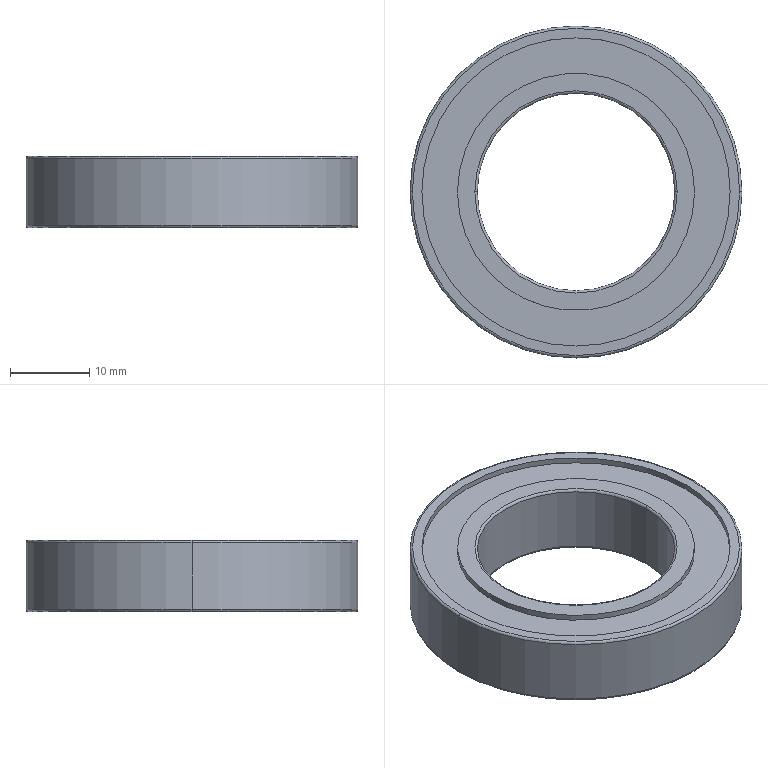Component | SolidWorks | BGRRB6905ZZ-1_bearingB6905ZZ-1 | 1 solid | 26 faces | box 42 x 42 x 9 mm | volume 7311 mm3 | cylinder 12 | torus 8 | plane 6 | commonest cylinder face diameters 39 x4 30 x4 42 x2 25 x2 | material AISI 1045 Steel, cold drawn
build123d program:
from build123d import *


with BuildPart() as part:
    # Sketch1 → Revolve1 (revolve)
    with BuildSketch(Plane.XY, mode=Mode.PRIVATE) as revolve1_sk:
        with BuildLine():
            Line((0, 20.7), (0, 19.5))
            Line((0, 19.5), (0.75, 19.5))
            Line((0.75, 19.5), (0.75, 15))
            Line((0.75, 15), (0, 15))
            Line((0, 15), (0, 12.8))
            ThreePointArc((0, 12.8), (0.08787, 12.588), (0.3, 12.5))
            Line((0.3, 12.5), (8.7, 12.5))
            ThreePointArc((8.7, 12.5), (8.912, 12.588), (9, 12.8))
            Line((9, 12.8), (9, 15))
            Line((9, 15), (8.25, 15))
            Line((8.25, 15), (8.25, 19.5))
            Line((8.25, 19.5), (9, 19.5))
            Line((9, 19.5), (9, 20.7))
            ThreePointArc((9, 20.7), (8.912, 20.912), (8.7, 21))
            Line((8.7, 21), (0.3, 21))
            ThreePointArc((0.3, 21), (0.08787, 20.912), (0, 20.7))
        make_face()
    revolve(revolve1_sk.sketch.rotate(Axis((9, 0, 0), (-1, 0, 0)), 270), axis=Axis((9, 0, 0), (-1, 0, 0)))


solid = part.part

# Placed as in the assembly
solid = solid.moved(Location((0, 0, 69), (0, 90, 0)))
STEP:
#1=COLOUR_RGB('',0.7922,0.8196,0.9333);
#2=FILL_AREA_STYLE_COLOUR('',#1);
#3=FILL_AREA_STYLE('',(#2));
#4=SURFACE_STYLE_FILL_AREA(#3);
#5=SURFACE_SIDE_STYLE('',(#4));
#6=SURFACE_STYLE_USAGE(.BOTH.,#5);
#7=PRESENTATION_STYLE_ASSIGNMENT((#6));
#8=CARTESIAN_POINT('',(-0.8268,0.,2.705));
#9=VERTEX_POINT('',#8);
#10=CARTESIAN_POINT('',(0.8268,0.,2.705));
#11=VERTEX_POINT('',#10);
#12=CARTESIAN_POINT('',(0.,0.,2.705));
#13=DIRECTION('',(0.,0.,-1.));
#14=DIRECTION('',(-1.,-0.,-0.));
#15=AXIS2_PLACEMENT_3D('',#12,#13,#14);
#16=CIRCLE('',#15,0.8268);
#17=EDGE_CURVE('',#9,#11,#16,.T.);
#18=ORIENTED_EDGE('',*,*,#17,.T.);
#19=CARTESIAN_POINT('',(0.8268,0.,2.374));
#20=VERTEX_POINT('',#19);
#21=CARTESIAN_POINT('',(0.8268,0.,2.717));
#22=DIRECTION('',(0.,0.,-1.));
#23=VECTOR('',#22,39.37);
#24=LINE('',#21,#23);
#25=EDGE_CURVE('',#11,#20,#24,.T.);
#26=ORIENTED_EDGE('',*,*,#25,.T.);
#27=CARTESIAN_POINT('',(-0.8268,0.,2.374));
#28=VERTEX_POINT('',#27);
#29=CARTESIAN_POINT('',(0.,0.,2.374));
#30=DIRECTION('',(0.,0.,-1.));
#31=DIRECTION('',(-1.,-0.,-0.));
#32=AXIS2_PLACEMENT_3D('',#29,#30,#31);
#33=CIRCLE('',#32,0.8268);
#34=EDGE_CURVE('',#28,#20,#33,.T.);
#35=ORIENTED_EDGE('',*,*,#34,.F.);
#36=CARTESIAN_POINT('',(-0.8268,0.,2.717));
#37=DIRECTION('',(0.,0.,-1.));
#38=VECTOR('',#37,39.37);
#39=LINE('',#36,#38);
#40=EDGE_CURVE('',#9,#28,#39,.T.);
#41=ORIENTED_EDGE('',*,*,#40,.F.);
#42=EDGE_LOOP('',(#18,#26,#35,#41));
#43=FACE_OUTER_BOUND('',#42,.T.);
#44=CARTESIAN_POINT('',(0.,0.,2.717));
#45=DIRECTION('',(0.,0.,-1.));
#46=DIRECTION('',(-1.,-0.,-0.));
#47=AXIS2_PLACEMENT_3D('',#44,#45,#46);
#48=CYLINDRICAL_SURFACE('',#47,0.8268);
#49=ADVANCED_FACE('',(#43),#48,.T.);
#50=CARTESIAN_POINT('',(-0.815,0.,2.717));
#51=VERTEX_POINT('',#50);
#52=CARTESIAN_POINT('',(0.815,0.,2.717));
#53=VERTEX_POINT('',#52);
#54=CARTESIAN_POINT('',(0.,0.,2.717));
#55=DIRECTION('',(0.,0.,-1.));
#56=DIRECTION('',(-1.,-0.,-0.));
#57=AXIS2_PLACEMENT_3D('',#54,#55,#56);
#58=CIRCLE('',#57,0.815);
#59=EDGE_CURVE('',#51,#53,#58,.T.);
#60=ORIENTED_EDGE('',*,*,#59,.T.);
#61=CARTESIAN_POINT('',(0.815,0.,2.705));
#62=DIRECTION('',(-0.,1.,0.));
#63=DIRECTION('',(-1.,-0.,0.));
#64=AXIS2_PLACEMENT_3D('',#61,#62,#63);
#65=CIRCLE('',#64,0.01181);
#66=EDGE_CURVE('',#53,#11,#65,.T.);
#67=ORIENTED_EDGE('',*,*,#66,.T.);
#68=ORIENTED_EDGE('',*,*,#17,.F.);
#69=CARTESIAN_POINT('',(-0.815,0.,2.705));
#70=DIRECTION('',(0.,-1.,-0.));
#71=DIRECTION('',(1.,0.,0.));
#72=AXIS2_PLACEMENT_3D('',#69,#70,#71);
#73=CIRCLE('',#72,0.01181);
#74=EDGE_CURVE('',#51,#9,#73,.T.);
#75=ORIENTED_EDGE('',*,*,#74,.F.);
#76=EDGE_LOOP('',(#60,#67,#68,#75));
#77=FACE_OUTER_BOUND('',#76,.T.);
#78=CARTESIAN_POINT('',(0.,0.,2.705));
#79=DIRECTION('',(0.,0.,-1.));
#80=DIRECTION('',(-1.,-0.,-0.));
#81=AXIS2_PLACEMENT_3D('',#78,#79,#80);
#82=TOROIDAL_SURFACE('',#81,0.815,0.01181);
#83=ADVANCED_FACE('',(#77),#82,.T.);
#84=CARTESIAN_POINT('',(0.7677,0.,2.717));
#85=VERTEX_POINT('',#84);
#86=CARTESIAN_POINT('',(-0.7677,0.,2.717));
#87=VERTEX_POINT('',#86);
#88=CARTESIAN_POINT('',(0.,0.,2.717));
#89=DIRECTION('',(0.,0.,-1.));
#90=DIRECTION('',(-1.,-0.,-0.));
#91=AXIS2_PLACEMENT_3D('',#88,#89,#90);
#92=CIRCLE('',#91,0.7677);
#93=EDGE_CURVE('',#85,#87,#92,.T.);
#94=ORIENTED_EDGE('',*,*,#93,.F.);
#95=CARTESIAN_POINT('',(0.7677,0.,2.687));
#96=VERTEX_POINT('',#95);
#97=CARTESIAN_POINT('',(0.7677,0.,2.717));
#98=DIRECTION('',(0.,0.,-1.));
#99=VECTOR('',#98,39.37);
#100=LINE('',#97,#99);
#101=EDGE_CURVE('',#85,#96,#100,.T.);
#102=ORIENTED_EDGE('',*,*,#101,.T.);
#103=CARTESIAN_POINT('',(-0.7677,0.,2.687));
#104=VERTEX_POINT('',#103);
#105=CARTESIAN_POINT('',(0.,0.,2.687));
#106=DIRECTION('',(0.,0.,-1.));
#107=DIRECTION('',(-1.,-0.,-0.));
#108=AXIS2_PLACEMENT_3D('',#105,#106,#107);
#109=CIRCLE('',#108,0.7677);
#110=EDGE_CURVE('',#96,#104,#109,.T.);
#111=ORIENTED_EDGE('',*,*,#110,.T.);
#112=CARTESIAN_POINT('',(-0.7677,0.,2.717));
#113=DIRECTION('',(0.,0.,-1.));
#114=VECTOR('',#113,39.37);
#115=LINE('',#112,#114);
#116=EDGE_CURVE('',#87,#104,#115,.T.);
#117=ORIENTED_EDGE('',*,*,#116,.F.);
#118=EDGE_LOOP('',(#94,#102,#111,#117));
#119=FACE_OUTER_BOUND('',#118,.T.);
#120=CARTESIAN_POINT('',(0.,0.,2.717));
#121=DIRECTION('',(0.,0.,-1.));
#122=DIRECTION('',(-1.,-0.,-0.));
#123=AXIS2_PLACEMENT_3D('',#120,#121,#122);
#124=CYLINDRICAL_SURFACE('',#123,0.7677);
#125=ADVANCED_FACE('',(#119),#124,.F.);
#126=CARTESIAN_POINT('',(-0.5906,0.,2.717));
#127=VERTEX_POINT('',#126);
#128=CARTESIAN_POINT('',(0.5906,0.,2.717));
#129=VERTEX_POINT('',#128);
#130=CARTESIAN_POINT('',(0.,0.,2.717));
#131=DIRECTION('',(0.,0.,-1.));
#132=DIRECTION('',(-1.,-0.,0.));
#133=AXIS2_PLACEMENT_3D('',#130,#131,#132);
#134=CIRCLE('',#133,0.5906);
#135=EDGE_CURVE('',#127,#129,#134,.T.);
#136=ORIENTED_EDGE('',*,*,#135,.T.);
#137=CARTESIAN_POINT('',(0.5906,0.,2.687));
#138=VERTEX_POINT('',#137);
#139=CARTESIAN_POINT('',(0.5906,0.,2.717));
#140=DIRECTION('',(0.,0.,-1.));
#141=VECTOR('',#140,39.37);
#142=LINE('',#139,#141);
#143=EDGE_CURVE('',#129,#138,#142,.T.);
#144=ORIENTED_EDGE('',*,*,#143,.T.);
#145=CARTESIAN_POINT('',(-0.5906,0.,2.687));
#146=VERTEX_POINT('',#145);
#147=CARTESIAN_POINT('',(0.,0.,2.687));
#148=DIRECTION('',(0.,0.,-1.));
#149=DIRECTION('',(-1.,-0.,0.));
#150=AXIS2_PLACEMENT_3D('',#147,#148,#149);
#151=CIRCLE('',#150,0.5906);
#152=EDGE_CURVE('',#146,#138,#151,.T.);
#153=ORIENTED_EDGE('',*,*,#152,.F.);
#154=CARTESIAN_POINT('',(-0.5906,0.,2.717));
#155=DIRECTION('',(0.,0.,-1.));
#156=VECTOR('',#155,39.37);
#157=LINE('',#154,#156);
#158=EDGE_CURVE('',#127,#146,#157,.T.);
#159=ORIENTED_EDGE('',*,*,#158,.F.);
#160=EDGE_LOOP('',(#136,#144,#153,#159));
#161=FACE_OUTER_BOUND('',#160,.T.);
#162=CARTESIAN_POINT('',(0.,0.,2.717));
#163=DIRECTION('',(0.,0.,-1.));
#164=DIRECTION('',(-1.,-0.,0.));
#165=AXIS2_PLACEMENT_3D('',#162,#163,#164);
#166=CYLINDRICAL_SURFACE('',#165,0.5906);
#167=ADVANCED_FACE('',(#161),#166,.T.);
#168=CARTESIAN_POINT('',(-0.4921,0.,2.705));
#169=VERTEX_POINT('',#168);
#170=CARTESIAN_POINT('',(0.4921,0.,2.705));
#171=VERTEX_POINT('',#170);
#172=CARTESIAN_POINT('',(0.,0.,2.705));
#173=DIRECTION('',(0.,0.,-1.));
#174=DIRECTION('',(-1.,-0.,0.));
#175=AXIS2_PLACEMENT_3D('',#172,#173,#174);
#176=CIRCLE('',#175,0.4921);
#177=EDGE_CURVE('',#169,#171,#176,.T.);
#178=ORIENTED_EDGE('',*,*,#177,.T.);
#179=CARTESIAN_POINT('',(0.5039,0.,2.717));
#180=VERTEX_POINT('',#179);
#181=CARTESIAN_POINT('',(0.5039,0.,2.705));
#182=DIRECTION('',(-0.,1.,0.));
#183=DIRECTION('',(-1.,-0.,0.));
#184=AXIS2_PLACEMENT_3D('',#181,#182,#183);
#185=CIRCLE('',#184,0.01181);
#186=EDGE_CURVE('',#171,#180,#185,.T.);
#187=ORIENTED_EDGE('',*,*,#186,.T.);
#188=CARTESIAN_POINT('',(-0.5039,0.,2.717));
#189=VERTEX_POINT('',#188);
#190=CARTESIAN_POINT('',(0.,0.,2.717));
#191=DIRECTION('',(0.,0.,-1.));
#192=DIRECTION('',(-1.,-0.,0.));
#193=AXIS2_PLACEMENT_3D('',#190,#191,#192);
#194=CIRCLE('',#193,0.5039);
#195=EDGE_CURVE('',#189,#180,#194,.T.);
#196=ORIENTED_EDGE('',*,*,#195,.F.);
#197=CARTESIAN_POINT('',(-0.5039,0.,2.705));
#198=DIRECTION('',(0.,-1.,-0.));
#199=DIRECTION('',(1.,0.,0.));
#200=AXIS2_PLACEMENT_3D('',#197,#198,#199);
#201=CIRCLE('',#200,0.01181);
#202=EDGE_CURVE('',#169,#189,#201,.T.);
#203=ORIENTED_EDGE('',*,*,#202,.F.);
#204=EDGE_LOOP('',(#178,#187,#196,#203));
#205=FACE_OUTER_BOUND('',#204,.T.);
#206=CARTESIAN_POINT('',(0.,0.,2.705));
#207=DIRECTION('',(0.,0.,-1.));
#208=DIRECTION('',(-1.,-0.,-0.));
#209=AXIS2_PLACEMENT_3D('',#206,#207,#208);
#210=TOROIDAL_SURFACE('',#209,0.5039,0.01181);
#211=ADVANCED_FACE('',(#205),#210,.T.);
#212=CARTESIAN_POINT('',(0.,0.,2.705));
#213=DIRECTION('',(0.,0.,-1.));
#214=DIRECTION('',(-1.,-0.,0.));
#215=AXIS2_PLACEMENT_3D('',#212,#213,#214);
#216=CIRCLE('',#215,0.4921);
#217=EDGE_CURVE('',#171,#169,#216,.T.);
#218=ORIENTED_EDGE('',*,*,#217,.F.);
#219=CARTESIAN_POINT('',(0.4921,0.,2.374));
#220=VERTEX_POINT('',#219);
#221=CARTESIAN_POINT('',(0.4921,0.,2.717));
#222=DIRECTION('',(0.,0.,-1.));
#223=VECTOR('',#222,39.37);
#224=LINE('',#221,#223);
#225=EDGE_CURVE('',#171,#220,#224,.T.);
#226=ORIENTED_EDGE('',*,*,#225,.T.);
#227=CARTESIAN_POINT('',(-0.4921,0.,2.374));
#228=VERTEX_POINT('',#227);
#229=CARTESIAN_POINT('',(0.,0.,2.374));
#230=DIRECTION('',(0.,0.,-1.));
#231=DIRECTION('',(-1.,-0.,-0.));
#232=AXIS2_PLACEMENT_3D('',#229,#230,#231);
#233=CIRCLE('',#232,0.4921);
#234=EDGE_CURVE('',#220,#228,#233,.T.);
#235=ORIENTED_EDGE('',*,*,#234,.T.);
#236=CARTESIAN_POINT('',(-0.4921,0.,2.717));
#237=DIRECTION('',(0.,0.,-1.));
#238=VECTOR('',#237,39.37);
#239=LINE('',#236,#238);
#240=EDGE_CURVE('',#169,#228,#239,.T.);
#241=ORIENTED_EDGE('',*,*,#240,.F.);
#242=EDGE_LOOP('',(#218,#226,#235,#241));
#243=FACE_OUTER_BOUND('',#242,.T.);
#244=CARTESIAN_POINT('',(0.,0.,2.717));
#245=DIRECTION('',(0.,0.,-1.));
#246=DIRECTION('',(-1.,-0.,0.));
#247=AXIS2_PLACEMENT_3D('',#244,#245,#246);
#248=CYLINDRICAL_SURFACE('',#247,0.4921);
#249=ADVANCED_FACE('',(#243),#248,.F.);
#250=CARTESIAN_POINT('',(-0.5039,0.,2.362));
#251=VERTEX_POINT('',#250);
#252=CARTESIAN_POINT('',(0.5039,0.,2.362));
#253=VERTEX_POINT('',#252);
#254=CARTESIAN_POINT('',(0.,0.,2.362));
#255=DIRECTION('',(0.,0.,-1.));
#256=DIRECTION('',(-1.,-0.,-0.));
#257=AXIS2_PLACEMENT_3D('',#254,#255,#256);
#258=CIRCLE('',#257,0.5039);
#259=EDGE_CURVE('',#251,#253,#258,.T.);
#260=ORIENTED_EDGE('',*,*,#259,.T.);
#261=CARTESIAN_POINT('',(0.5039,0.,2.374));
#262=DIRECTION('',(-0.,1.,0.));
#263=DIRECTION('',(-1.,-0.,0.));
#264=AXIS2_PLACEMENT_3D('',#261,#262,#263);
#265=CIRCLE('',#264,0.01181);
#266=EDGE_CURVE('',#253,#220,#265,.T.);
#267=ORIENTED_EDGE('',*,*,#266,.T.);
#268=CARTESIAN_POINT('',(0.,0.,2.374));
#269=DIRECTION('',(0.,0.,-1.));
#270=DIRECTION('',(-1.,-0.,-0.));
#271=AXIS2_PLACEMENT_3D('',#268,#269,#270);
#272=CIRCLE('',#271,0.4921);
#273=EDGE_CURVE('',#228,#220,#272,.T.);
#274=ORIENTED_EDGE('',*,*,#273,.F.);
#275=CARTESIAN_POINT('',(-0.5039,0.,2.374));
#276=DIRECTION('',(0.,-1.,-0.));
#277=DIRECTION('',(1.,0.,0.));
#278=AXIS2_PLACEMENT_3D('',#275,#276,#277);
#279=CIRCLE('',#278,0.01181);
#280=EDGE_CURVE('',#251,#228,#279,.T.);
#281=ORIENTED_EDGE('',*,*,#280,.F.);
#282=EDGE_LOOP('',(#260,#267,#274,#281));
#283=FACE_OUTER_BOUND('',#282,.T.);
#284=CARTESIAN_POINT('',(0.,0.,2.374));
#285=DIRECTION('',(0.,0.,-1.));
#286=DIRECTION('',(-1.,-0.,-0.));
#287=AXIS2_PLACEMENT_3D('',#284,#285,#286);
#288=TOROIDAL_SURFACE('',#287,0.5039,0.01181);
#289=ADVANCED_FACE('',(#283),#288,.T.);
#290=CARTESIAN_POINT('',(-0.5906,0.,2.392));
#291=VERTEX_POINT('',#290);
#292=CARTESIAN_POINT('',(0.5906,0.,2.392));
#293=VERTEX_POINT('',#292);
#294=CARTESIAN_POINT('',(0.,0.,2.392));
#295=DIRECTION('',(0.,0.,-1.));
#296=DIRECTION('',(-1.,-0.,-0.));
#297=AXIS2_PLACEMENT_3D('',#294,#295,#296);
#298=CIRCLE('',#297,0.5906);
#299=EDGE_CURVE('',#291,#293,#298,.T.);
#300=ORIENTED_EDGE('',*,*,#299,.T.);
#301=CARTESIAN_POINT('',(0.5906,0.,2.362));
#302=VERTEX_POINT('',#301);
#303=CARTESIAN_POINT('',(0.5906,0.,2.717));
#304=DIRECTION('',(0.,0.,-1.));
#305=VECTOR('',#304,39.37);
#306=LINE('',#303,#305);
#307=EDGE_CURVE('',#293,#302,#306,.T.);
#308=ORIENTED_EDGE('',*,*,#307,.T.);
#309=CARTESIAN_POINT('',(-0.5906,0.,2.362));
#310=VERTEX_POINT('',#309);
#311=CARTESIAN_POINT('',(0.,0.,2.362));
#312=DIRECTION('',(0.,0.,-1.));
#313=DIRECTION('',(-1.,-0.,-0.));
#314=AXIS2_PLACEMENT_3D('',#311,#312,#313);
#315=CIRCLE('',#314,0.5906);
#316=EDGE_CURVE('',#310,#302,#315,.T.);
#317=ORIENTED_EDGE('',*,*,#316,.F.);
#318=CARTESIAN_POINT('',(-0.5906,0.,2.717));
#319=DIRECTION('',(0.,0.,-1.));
#320=VECTOR('',#319,39.37);
#321=LINE('',#318,#320);
#322=EDGE_CURVE('',#291,#310,#321,.T.);
#323=ORIENTED_EDGE('',*,*,#322,.F.);
#324=EDGE_LOOP('',(#300,#308,#317,#323));
#325=FACE_OUTER_BOUND('',#324,.T.);
#326=CARTESIAN_POINT('',(0.,0.,2.717));
#327=DIRECTION('',(0.,0.,-1.));
#328=DIRECTION('',(-1.,-0.,0.));
#329=AXIS2_PLACEMENT_3D('',#326,#327,#328);
#330=CYLINDRICAL_SURFACE('',#329,0.5906);
#331=ADVANCED_FACE('',(#325),#330,.T.);
#332=CARTESIAN_POINT('',(0.7677,0.,2.392));
#333=VERTEX_POINT('',#332);
#334=CARTESIAN_POINT('',(-0.7677,0.,2.392));
#335=VERTEX_POINT('',#334);
#336=CARTESIAN_POINT('',(0.,0.,2.392));
#337=DIRECTION('',(0.,0.,-1.));
#338=DIRECTION('',(-1.,-0.,-0.));
#339=AXIS2_PLACEMENT_3D('',#336,#337,#338);
#340=CIRCLE('',#339,0.7677);
#341=EDGE_CURVE('',#333,#335,#340,.T.);
#342=ORIENTED_EDGE('',*,*,#341,.F.);
#343=CARTESIAN_POINT('',(0.7677,0.,2.362));
#344=VERTEX_POINT('',#343);
#345=CARTESIAN_POINT('',(0.7677,0.,2.717));
#346=DIRECTION('',(0.,0.,-1.));
#347=VECTOR('',#346,39.37);
#348=LINE('',#345,#347);
#349=EDGE_CURVE('',#333,#344,#348,.T.);
#350=ORIENTED_EDGE('',*,*,#349,.T.);
#351=CARTESIAN_POINT('',(-0.7677,0.,2.362));
#352=VERTEX_POINT('',#351);
#353=CARTESIAN_POINT('',(0.,0.,2.362));
#354=DIRECTION('',(0.,0.,-1.));
#355=DIRECTION('',(-1.,-0.,-0.));
#356=AXIS2_PLACEMENT_3D('',#353,#354,#355);
#357=CIRCLE('',#356,0.7677);
#358=EDGE_CURVE('',#344,#352,#357,.T.);
#359=ORIENTED_EDGE('',*,*,#358,.T.);
#360=CARTESIAN_POINT('',(-0.7677,0.,2.717));
#361=DIRECTION('',(0.,0.,-1.));
#362=VECTOR('',#361,39.37);
#363=LINE('',#360,#362);
#364=EDGE_CURVE('',#335,#352,#363,.T.);
#365=ORIENTED_EDGE('',*,*,#364,.F.);
#366=EDGE_LOOP('',(#342,#350,#359,#365));
#367=FACE_OUTER_BOUND('',#366,.T.);
#368=CARTESIAN_POINT('',(0.,0.,2.717));
#369=DIRECTION('',(0.,0.,-1.));
#370=DIRECTION('',(-1.,-0.,-0.));
#371=AXIS2_PLACEMENT_3D('',#368,#369,#370);
#372=CYLINDRICAL_SURFACE('',#371,0.7677);
#373=ADVANCED_FACE('',(#367),#372,.F.);
#374=ORIENTED_EDGE('',*,*,#34,.T.);
#375=CARTESIAN_POINT('',(0.815,0.,2.362));
#376=VERTEX_POINT('',#375);
#377=CARTESIAN_POINT('',(0.815,0.,2.374));
#378=DIRECTION('',(-0.,1.,0.));
#379=DIRECTION('',(-1.,-0.,0.));
#380=AXIS2_PLACEMENT_3D('',#377,#378,#379);
#381=CIRCLE('',#380,0.01181);
#382=EDGE_CURVE('',#20,#376,#381,.T.);
#383=ORIENTED_EDGE('',*,*,#382,.T.);
#384=CARTESIAN_POINT('',(-0.815,0.,2.362));
#385=VERTEX_POINT('',#384);
#386=CARTESIAN_POINT('',(0.,0.,2.362));
#387=DIRECTION('',(0.,0.,-1.));
#388=DIRECTION('',(-1.,-0.,-0.));
#389=AXIS2_PLACEMENT_3D('',#386,#387,#388);
#390=CIRCLE('',#389,0.815);
#391=EDGE_CURVE('',#385,#376,#390,.T.);
#392=ORIENTED_EDGE('',*,*,#391,.F.);
#393=CARTESIAN_POINT('',(-0.815,0.,2.374));
#394=DIRECTION('',(0.,-1.,-0.));
#395=DIRECTION('',(1.,0.,0.));
#396=AXIS2_PLACEMENT_3D('',#393,#394,#395);
#397=CIRCLE('',#396,0.01181);
#398=EDGE_CURVE('',#28,#385,#397,.T.);
#399=ORIENTED_EDGE('',*,*,#398,.F.);
#400=EDGE_LOOP('',(#374,#383,#392,#399));
#401=FACE_OUTER_BOUND('',#400,.T.);
#402=CARTESIAN_POINT('',(0.,0.,2.374));
#403=DIRECTION('',(0.,0.,-1.));
#404=DIRECTION('',(-1.,-0.,-0.));
#405=AXIS2_PLACEMENT_3D('',#402,#403,#404);
#406=TOROIDAL_SURFACE('',#405,0.815,0.01181);
#407=ADVANCED_FACE('',(#401),#406,.T.);
#408=ORIENTED_EDGE('',*,*,#382,.F.);
#409=CARTESIAN_POINT('',(0.,0.,2.374));
#410=DIRECTION('',(0.,0.,-1.));
#411=DIRECTION('',(-1.,-0.,-0.));
#412=AXIS2_PLACEMENT_3D('',#409,#410,#411);
#413=CIRCLE('',#412,0.8268);
#414=EDGE_CURVE('',#20,#28,#413,.T.);
#415=ORIENTED_EDGE('',*,*,#414,.T.);
#416=ORIENTED_EDGE('',*,*,#398,.T.);
#417=CARTESIAN_POINT('',(0.,0.,2.362));
#418=DIRECTION('',(0.,0.,-1.));
#419=DIRECTION('',(-1.,-0.,-0.));
#420=AXIS2_PLACEMENT_3D('',#417,#418,#419);
#421=CIRCLE('',#420,0.815);
#422=EDGE_CURVE('',#376,#385,#421,.T.);
#423=ORIENTED_EDGE('',*,*,#422,.F.);
#424=EDGE_LOOP('',(#408,#415,#416,#423));
#425=FACE_OUTER_BOUND('',#424,.T.);
#426=CARTESIAN_POINT('',(0.,0.,2.374));
#427=DIRECTION('',(0.,0.,-1.));
#428=DIRECTION('',(-1.,-0.,-0.));
#429=AXIS2_PLACEMENT_3D('',#426,#427,#428);
#430=TOROIDAL_SURFACE('',#429,0.815,0.01181);
#431=ADVANCED_FACE('',(#425),#430,.T.);
#432=CARTESIAN_POINT('',(0.,0.,2.362));
#433=DIRECTION('',(0.,0.,-1.));
#434=DIRECTION('',(-1.,-0.,-0.));
#435=AXIS2_PLACEMENT_3D('',#432,#433,#434);
#436=CIRCLE('',#435,0.7677);
#437=EDGE_CURVE('',#352,#344,#436,.T.);
#438=ORIENTED_EDGE('',*,*,#437,.F.);
#439=ORIENTED_EDGE('',*,*,#358,.F.);
#440=EDGE_LOOP('',(#438,#439));
#441=FACE_BOUND('',#440,.T.);
#442=ORIENTED_EDGE('',*,*,#391,.T.);
#443=ORIENTED_EDGE('',*,*,#422,.T.);
#444=EDGE_LOOP('',(#442,#443));
#445=FACE_OUTER_BOUND('',#444,.T.);
#446=CARTESIAN_POINT('',(0.,0.815,2.362));
#447=DIRECTION('',(-0.,-0.,1.));
#448=DIRECTION('',(1.,0.,0.));
#449=AXIS2_PLACEMENT_3D('',#446,#447,#448);
#450=PLANE('',#449);
#451=ADVANCED_FACE('',(#441,#445),#450,.F.);
#452=ORIENTED_EDGE('',*,*,#349,.F.);
#453=CARTESIAN_POINT('',(0.,0.,2.392));
#454=DIRECTION('',(0.,0.,-1.));
#455=DIRECTION('',(-1.,-0.,-0.));
#456=AXIS2_PLACEMENT_3D('',#453,#454,#455);
#457=CIRCLE('',#456,0.7677);
#458=EDGE_CURVE('',#335,#333,#457,.T.);
#459=ORIENTED_EDGE('',*,*,#458,.F.);
#460=ORIENTED_EDGE('',*,*,#364,.T.);
#461=ORIENTED_EDGE('',*,*,#437,.T.);
#462=EDGE_LOOP('',(#452,#459,#460,#461));
#463=FACE_OUTER_BOUND('',#462,.T.);
#464=CARTESIAN_POINT('',(0.,0.,2.717));
#465=DIRECTION('',(0.,0.,-1.));
#466=DIRECTION('',(-1.,-0.,-0.));
#467=AXIS2_PLACEMENT_3D('',#464,#465,#466);
#468=CYLINDRICAL_SURFACE('',#467,0.7677);
#469=ADVANCED_FACE('',(#463),#468,.F.);
#470=ORIENTED_EDGE('',*,*,#299,.F.);
#471=CARTESIAN_POINT('',(0.,0.,2.392));
#472=DIRECTION('',(0.,0.,-1.));
#473=DIRECTION('',(-1.,-0.,-0.));
#474=AXIS2_PLACEMENT_3D('',#471,#472,#473);
#475=CIRCLE('',#474,0.5906);
#476=EDGE_CURVE('',#293,#291,#475,.T.);
#477=ORIENTED_EDGE('',*,*,#476,.F.);
#478=EDGE_LOOP('',(#470,#477));
#479=FACE_BOUND('',#478,.T.);
#480=ORIENTED_EDGE('',*,*,#458,.T.);
#481=ORIENTED_EDGE('',*,*,#341,.T.);
#482=EDGE_LOOP('',(#480,#481));
#483=FACE_OUTER_BOUND('',#482,.T.);
#484=CARTESIAN_POINT('',(0.,0.7677,2.392));
#485=DIRECTION('',(-0.,-0.,1.));
#486=DIRECTION('',(1.,0.,0.));
#487=AXIS2_PLACEMENT_3D('',#484,#485,#486);
#488=PLANE('',#487);
#489=ADVANCED_FACE('',(#479,#483),#488,.F.);
#490=ORIENTED_EDGE('',*,*,#307,.F.);
#491=ORIENTED_EDGE('',*,*,#476,.T.);
#492=ORIENTED_EDGE('',*,*,#322,.T.);
#493=CARTESIAN_POINT('',(0.,0.,2.362));
#494=DIRECTION('',(0.,0.,-1.));
#495=DIRECTION('',(-1.,-0.,-0.));
#496=AXIS2_PLACEMENT_3D('',#493,#494,#495);
#497=CIRCLE('',#496,0.5906);
#498=EDGE_CURVE('',#302,#310,#497,.T.);
#499=ORIENTED_EDGE('',*,*,#498,.F.);
#500=EDGE_LOOP('',(#490,#491,#492,#499));
#501=FACE_OUTER_BOUND('',#500,.T.);
#502=CARTESIAN_POINT('',(0.,0.,2.717));
#503=DIRECTION('',(0.,0.,-1.));
#504=DIRECTION('',(-1.,-0.,0.));
#505=AXIS2_PLACEMENT_3D('',#502,#503,#504);
#506=CYLINDRICAL_SURFACE('',#505,0.5906);
#507=ADVANCED_FACE('',(#501),#506,.T.);
#508=ORIENTED_EDGE('',*,*,#259,.F.);
#509=CARTESIAN_POINT('',(0.,0.,2.362));
#510=DIRECTION('',(0.,0.,-1.));
#511=DIRECTION('',(-1.,-0.,-0.));
#512=AXIS2_PLACEMENT_3D('',#509,#510,#511);
#513=CIRCLE('',#512,0.5039);
#514=EDGE_CURVE('',#253,#251,#513,.T.);
#515=ORIENTED_EDGE('',*,*,#514,.F.);
#516=EDGE_LOOP('',(#508,#515));
#517=FACE_BOUND('',#516,.T.);
#518=ORIENTED_EDGE('',*,*,#316,.T.);
#519=ORIENTED_EDGE('',*,*,#498,.T.);
#520=EDGE_LOOP('',(#518,#519));
#521=FACE_OUTER_BOUND('',#520,.T.);
#522=CARTESIAN_POINT('',(0.,0.5906,2.362));
#523=DIRECTION('',(-0.,-0.,1.));
#524=DIRECTION('',(1.,0.,0.));
#525=AXIS2_PLACEMENT_3D('',#522,#523,#524);
#526=PLANE('',#525);
#527=ADVANCED_FACE('',(#517,#521),#526,.F.);
#528=ORIENTED_EDGE('',*,*,#266,.F.);
#529=ORIENTED_EDGE('',*,*,#514,.T.);
#530=ORIENTED_EDGE('',*,*,#280,.T.);
#531=ORIENTED_EDGE('',*,*,#234,.F.);
#532=EDGE_LOOP('',(#528,#529,#530,#531));
#533=FACE_OUTER_BOUND('',#532,.T.);
#534=CARTESIAN_POINT('',(0.,0.,2.374));
#535=DIRECTION('',(0.,0.,-1.));
#536=DIRECTION('',(-1.,-0.,-0.));
#537=AXIS2_PLACEMENT_3D('',#534,#535,#536);
#538=TOROIDAL_SURFACE('',#537,0.5039,0.01181);
#539=ADVANCED_FACE('',(#533),#538,.T.);
#540=ORIENTED_EDGE('',*,*,#225,.F.);
#541=ORIENTED_EDGE('',*,*,#177,.F.);
#542=ORIENTED_EDGE('',*,*,#240,.T.);
#543=ORIENTED_EDGE('',*,*,#273,.T.);
#544=EDGE_LOOP('',(#540,#541,#542,#543));
#545=FACE_OUTER_BOUND('',#544,.T.);
#546=CARTESIAN_POINT('',(0.,0.,2.717));
#547=DIRECTION('',(0.,0.,-1.));
#548=DIRECTION('',(-1.,-0.,0.));
#549=AXIS2_PLACEMENT_3D('',#546,#547,#548);
#550=CYLINDRICAL_SURFACE('',#549,0.4921);
#551=ADVANCED_FACE('',(#545),#550,.F.);
#552=ORIENTED_EDGE('',*,*,#186,.F.);
#553=ORIENTED_EDGE('',*,*,#217,.T.);
#554=ORIENTED_EDGE('',*,*,#202,.T.);
#555=CARTESIAN_POINT('',(0.,0.,2.717));
#556=DIRECTION('',(0.,0.,-1.));
#557=DIRECTION('',(-1.,-0.,0.));
#558=AXIS2_PLACEMENT_3D('',#555,#556,#557);
#559=CIRCLE('',#558,0.5039);
#560=EDGE_CURVE('',#180,#189,#559,.T.);
#561=ORIENTED_EDGE('',*,*,#560,.F.);
#562=EDGE_LOOP('',(#552,#553,#554,#561));
#563=FACE_OUTER_BOUND('',#562,.T.);
#564=CARTESIAN_POINT('',(0.,0.,2.705));
#565=DIRECTION('',(0.,0.,-1.));
#566=DIRECTION('',(-1.,-0.,-0.));
#567=AXIS2_PLACEMENT_3D('',#564,#565,#566);
#568=TOROIDAL_SURFACE('',#567,0.5039,0.01181);
#569=ADVANCED_FACE('',(#563),#568,.T.);
#570=ORIENTED_EDGE('',*,*,#135,.F.);
#571=CARTESIAN_POINT('',(0.,0.,2.717));
#572=DIRECTION('',(0.,0.,-1.));
#573=DIRECTION('',(-1.,-0.,0.));
#574=AXIS2_PLACEMENT_3D('',#571,#572,#573);
#575=CIRCLE('',#574,0.5906);
#576=EDGE_CURVE('',#129,#127,#575,.T.);
#577=ORIENTED_EDGE('',*,*,#576,.F.);
#578=EDGE_LOOP('',(#570,#577));
#579=FACE_OUTER_BOUND('',#578,.T.);
#580=ORIENTED_EDGE('',*,*,#195,.T.);
#581=ORIENTED_EDGE('',*,*,#560,.T.);
#582=EDGE_LOOP('',(#580,#581));
#583=FACE_BOUND('',#582,.T.);
#584=CARTESIAN_POINT('',(0.,0.5039,2.717));
#585=DIRECTION('',(0.,0.,-1.));
#586=DIRECTION('',(-1.,-0.,-0.));
#587=AXIS2_PLACEMENT_3D('',#584,#585,#586);
#588=PLANE('',#587);
#589=ADVANCED_FACE('',(#579,#583),#588,.F.);
#590=ORIENTED_EDGE('',*,*,#143,.F.);
#591=ORIENTED_EDGE('',*,*,#576,.T.);
#592=ORIENTED_EDGE('',*,*,#158,.T.);
#593=CARTESIAN_POINT('',(0.,0.,2.687));
#594=DIRECTION('',(0.,0.,-1.));
#595=DIRECTION('',(-1.,-0.,0.));
#596=AXIS2_PLACEMENT_3D('',#593,#594,#595);
#597=CIRCLE('',#596,0.5906);
#598=EDGE_CURVE('',#138,#146,#597,.T.);
#599=ORIENTED_EDGE('',*,*,#598,.F.);
#600=EDGE_LOOP('',(#590,#591,#592,#599));
#601=FACE_OUTER_BOUND('',#600,.T.);
#602=CARTESIAN_POINT('',(0.,0.,2.717));
#603=DIRECTION('',(0.,0.,-1.));
#604=DIRECTION('',(-1.,-0.,0.));
#605=AXIS2_PLACEMENT_3D('',#602,#603,#604);
#606=CYLINDRICAL_SURFACE('',#605,0.5906);
#607=ADVANCED_FACE('',(#601),#606,.T.);
#608=CARTESIAN_POINT('',(0.,0.,2.687));
#609=DIRECTION('',(0.,0.,-1.));
#610=DIRECTION('',(-1.,-0.,-0.));
#611=AXIS2_PLACEMENT_3D('',#608,#609,#610);
#612=CIRCLE('',#611,0.7677);
#613=EDGE_CURVE('',#104,#96,#612,.T.);
#614=ORIENTED_EDGE('',*,*,#613,.F.);
#615=ORIENTED_EDGE('',*,*,#110,.F.);
#616=EDGE_LOOP('',(#614,#615));
#617=FACE_OUTER_BOUND('',#616,.T.);
#618=ORIENTED_EDGE('',*,*,#152,.T.);
#619=ORIENTED_EDGE('',*,*,#598,.T.);
#620=EDGE_LOOP('',(#618,#619));
#621=FACE_BOUND('',#620,.T.);
#622=CARTESIAN_POINT('',(0.,0.5906,2.687));
#623=DIRECTION('',(0.,0.,-1.));
#624=DIRECTION('',(-1.,-0.,-0.));
#625=AXIS2_PLACEMENT_3D('',#622,#623,#624);
#626=PLANE('',#625);
#627=ADVANCED_FACE('',(#617,#621),#626,.F.);
#628=ORIENTED_EDGE('',*,*,#101,.F.);
#629=CARTESIAN_POINT('',(0.,0.,2.717));
#630=DIRECTION('',(0.,0.,-1.));
#631=DIRECTION('',(-1.,-0.,-0.));
#632=AXIS2_PLACEMENT_3D('',#629,#630,#631);
#633=CIRCLE('',#632,0.7677);
#634=EDGE_CURVE('',#87,#85,#633,.T.);
#635=ORIENTED_EDGE('',*,*,#634,.F.);
#636=ORIENTED_EDGE('',*,*,#116,.T.);
#637=ORIENTED_EDGE('',*,*,#613,.T.);
#638=EDGE_LOOP('',(#628,#635,#636,#637));
#639=FACE_OUTER_BOUND('',#638,.T.);
#640=CARTESIAN_POINT('',(0.,0.,2.717));
#641=DIRECTION('',(0.,0.,-1.));
#642=DIRECTION('',(-1.,-0.,-0.));
#643=AXIS2_PLACEMENT_3D('',#640,#641,#642);
#644=CYLINDRICAL_SURFACE('',#643,0.7677);
#645=ADVANCED_FACE('',(#639),#644,.F.);
#646=ORIENTED_EDGE('',*,*,#59,.F.);
#647=CARTESIAN_POINT('',(0.,0.,2.717));
#648=DIRECTION('',(0.,0.,-1.));
#649=DIRECTION('',(-1.,-0.,-0.));
#650=AXIS2_PLACEMENT_3D('',#647,#648,#649);
#651=CIRCLE('',#650,0.815);
#652=EDGE_CURVE('',#53,#51,#651,.T.);
#653=ORIENTED_EDGE('',*,*,#652,.F.);
#654=EDGE_LOOP('',(#646,#653));
#655=FACE_OUTER_BOUND('',#654,.T.);
#656=ORIENTED_EDGE('',*,*,#634,.T.);
#657=ORIENTED_EDGE('',*,*,#93,.T.);
#658=EDGE_LOOP('',(#656,#657));
#659=FACE_BOUND('',#658,.T.);
#660=CARTESIAN_POINT('',(0.,0.7677,2.717));
#661=DIRECTION('',(0.,0.,-1.));
#662=DIRECTION('',(-1.,-0.,-0.));
#663=AXIS2_PLACEMENT_3D('',#660,#661,#662);
#664=PLANE('',#663);
#665=ADVANCED_FACE('',(#655,#659),#664,.F.);
#666=ORIENTED_EDGE('',*,*,#66,.F.);
#667=ORIENTED_EDGE('',*,*,#652,.T.);
#668=ORIENTED_EDGE('',*,*,#74,.T.);
#669=CARTESIAN_POINT('',(0.,0.,2.705));
#670=DIRECTION('',(0.,0.,-1.));
#671=DIRECTION('',(-1.,-0.,-0.));
#672=AXIS2_PLACEMENT_3D('',#669,#670,#671);
#673=CIRCLE('',#672,0.8268);
#674=EDGE_CURVE('',#11,#9,#673,.T.);
#675=ORIENTED_EDGE('',*,*,#674,.F.);
#676=EDGE_LOOP('',(#666,#667,#668,#675));
#677=FACE_OUTER_BOUND('',#676,.T.);
#678=CARTESIAN_POINT('',(0.,0.,2.705));
#679=DIRECTION('',(0.,0.,-1.));
#680=DIRECTION('',(-1.,-0.,-0.));
#681=AXIS2_PLACEMENT_3D('',#678,#679,#680);
#682=TOROIDAL_SURFACE('',#681,0.815,0.01181);
#683=ADVANCED_FACE('',(#677),#682,.T.);
#684=ORIENTED_EDGE('',*,*,#25,.F.);
#685=ORIENTED_EDGE('',*,*,#674,.T.);
#686=ORIENTED_EDGE('',*,*,#40,.T.);
#687=ORIENTED_EDGE('',*,*,#414,.F.);
#688=EDGE_LOOP('',(#684,#685,#686,#687));
#689=FACE_OUTER_BOUND('',#688,.T.);
#690=CARTESIAN_POINT('',(0.,0.,2.717));
#691=DIRECTION('',(0.,0.,-1.));
#692=DIRECTION('',(-1.,-0.,-0.));
#693=AXIS2_PLACEMENT_3D('',#690,#691,#692);
#694=CYLINDRICAL_SURFACE('',#693,0.8268);
#695=ADVANCED_FACE('',(#689),#694,.T.);
#696=CLOSED_SHELL('',(#49,#83,#125,#167,#211,#249,#289,#331,#373,#407,#431,#451,#469,#489,#507,#527,#539,#551,#569,#589,#607,#627,#645,#665,#683,#695));
#697=MANIFOLD_SOLID_BREP('',#696);
#698=STYLED_ITEM('',(#7),#697);
#699=PRESENTATION_LAYER_ASSIGNMENT('','',(#698));
#700=(LENGTH_UNIT()NAMED_UNIT(*)SI_UNIT($,.METRE.));
#701=LENGTH_MEASURE_WITH_UNIT(LENGTH_MEASURE(0.0254),#700);
#702=DIMENSIONAL_EXPONENTS(1.,0.,0.,0.,0.,0.,0.);
#703=(CONVERSION_BASED_UNIT('',#701)LENGTH_UNIT()NAMED_UNIT(#702));
#704=UNCERTAINTY_MEASURE_WITH_UNIT(LENGTH_MEASURE(0.00001),#703,'','');
#705=(NAMED_UNIT(*)PLANE_ANGLE_UNIT()SI_UNIT($,.RADIAN.));
#706=(NAMED_UNIT(*)SI_UNIT($,.STERADIAN.)SOLID_ANGLE_UNIT());
#707=(GEOMETRIC_REPRESENTATION_CONTEXT(3)GLOBAL_UNCERTAINTY_ASSIGNED_CONTEXT((#704))GLOBAL_UNIT_ASSIGNED_CONTEXT((#703,#705,#706))REPRESENTATION_CONTEXT('',''));
#708=MECHANICAL_DESIGN_GEOMETRIC_PRESENTATION_REPRESENTATION('',(#698),#707);
#709=CARTESIAN_POINT('',(0.,0.,0.));
#710=DIRECTION('',(0.,0.,1.));
#711=DIRECTION('',(1.,0.,0.));
#712=AXIS2_PLACEMENT_3D('',#709,#710,#711);
#713=(LENGTH_UNIT()NAMED_UNIT(*)SI_UNIT($,.METRE.));
#714=LENGTH_MEASURE_WITH_UNIT(LENGTH_MEASURE(0.0254),#713);
#715=DIMENSIONAL_EXPONENTS(1.,0.,0.,0.,0.,0.,0.);
#716=(CONVERSION_BASED_UNIT('',#714)LENGTH_UNIT()NAMED_UNIT(#715));
#717=UNCERTAINTY_MEASURE_WITH_UNIT(LENGTH_MEASURE(0.00001),#716,'','');
#718=(NAMED_UNIT(*)PLANE_ANGLE_UNIT()SI_UNIT($,.RADIAN.));
#719=(NAMED_UNIT(*)SI_UNIT($,.STERADIAN.)SOLID_ANGLE_UNIT());
#720=(GEOMETRIC_REPRESENTATION_CONTEXT(3)GLOBAL_UNCERTAINTY_ASSIGNED_CONTEXT((#717))GLOBAL_UNIT_ASSIGNED_CONTEXT((#716,#718,#719))REPRESENTATION_CONTEXT('',''));
#721=ADVANCED_BREP_SHAPE_REPRESENTATION('',(#697,#712),#720);